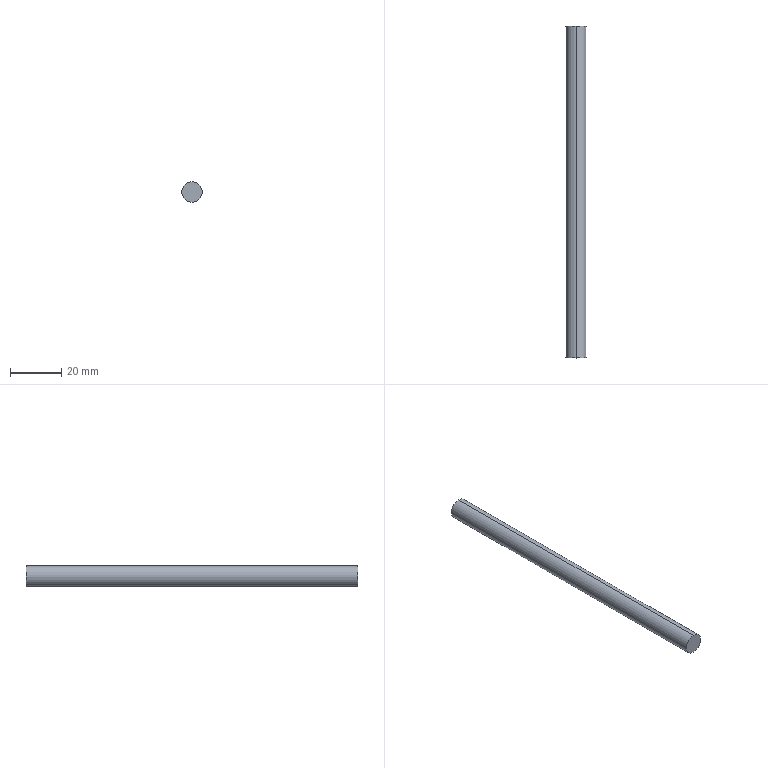Component | SolidWorks | LeadScrewM8x130-1 | 1 solid | 4 faces | box 8 x 130 x 8 mm | volume 6535 mm3 | cylinder 2 | plane 2 | commonest cylinder face diameters 8 x2
STEP:
#1=COLOUR_RGB('',0.7922,0.8196,0.9333);
#2=FILL_AREA_STYLE_COLOUR('',#1);
#3=FILL_AREA_STYLE('',(#2));
#4=SURFACE_STYLE_FILL_AREA(#3);
#5=SURFACE_SIDE_STYLE('',(#4));
#6=SURFACE_STYLE_USAGE(.BOTH.,#5);
#7=PRESENTATION_STYLE_ASSIGNMENT((#6));
#8=CARTESIAN_POINT('',(240.374,117.231,2.023));
#9=VERTEX_POINT('',#8);
#10=CARTESIAN_POINT('',(240.374,117.231,1.708));
#11=VERTEX_POINT('',#10);
#12=CARTESIAN_POINT('',(240.374,117.231,1.865));
#13=DIRECTION('',(0.,1.,-0.));
#14=DIRECTION('',(0.,0.,-1.));
#15=AXIS2_PLACEMENT_3D('',#12,#13,#14);
#16=CIRCLE('',#15,0.1575);
#17=EDGE_CURVE('',#9,#11,#16,.T.);
#18=ORIENTED_EDGE('',*,*,#17,.T.);
#19=CARTESIAN_POINT('',(240.374,122.35,1.708));
#20=VERTEX_POINT('',#19);
#21=CARTESIAN_POINT('',(240.374,118.413,1.708));
#22=DIRECTION('',(0.,1.,-0.));
#23=VECTOR('',#22,39.37);
#24=LINE('',#21,#23);
#25=EDGE_CURVE('',#11,#20,#24,.T.);
#26=ORIENTED_EDGE('',*,*,#25,.T.);
#27=CARTESIAN_POINT('',(240.374,122.35,2.023));
#28=VERTEX_POINT('',#27);
#29=CARTESIAN_POINT('',(240.374,122.35,1.865));
#30=DIRECTION('',(-0.,-1.,0.));
#31=DIRECTION('',(0.,0.,-1.));
#32=AXIS2_PLACEMENT_3D('',#29,#30,#31);
#33=CIRCLE('',#32,0.1575);
#34=EDGE_CURVE('',#20,#28,#33,.T.);
#35=ORIENTED_EDGE('',*,*,#34,.T.);
#36=CARTESIAN_POINT('',(240.374,118.413,2.023));
#37=DIRECTION('',(0.,1.,-0.));
#38=VECTOR('',#37,39.37);
#39=LINE('',#36,#38);
#40=EDGE_CURVE('',#9,#28,#39,.T.);
#41=ORIENTED_EDGE('',*,*,#40,.F.);
#42=EDGE_LOOP('',(#18,#26,#35,#41));
#43=FACE_OUTER_BOUND('',#42,.T.);
#44=CARTESIAN_POINT('',(240.374,118.413,1.865));
#45=DIRECTION('',(0.,1.,-0.));
#46=DIRECTION('',(0.,0.,1.));
#47=AXIS2_PLACEMENT_3D('',#44,#45,#46);
#48=CYLINDRICAL_SURFACE('',#47,0.1575);
#49=ADVANCED_FACE('',(#43),#48,.T.);
#50=CARTESIAN_POINT('',(240.374,122.35,1.865));
#51=DIRECTION('',(-0.,-1.,0.));
#52=DIRECTION('',(0.,0.,-1.));
#53=AXIS2_PLACEMENT_3D('',#50,#51,#52);
#54=CIRCLE('',#53,0.1575);
#55=EDGE_CURVE('',#28,#20,#54,.T.);
#56=ORIENTED_EDGE('',*,*,#55,.F.);
#57=ORIENTED_EDGE('',*,*,#34,.F.);
#58=EDGE_LOOP('',(#56,#57));
#59=FACE_OUTER_BOUND('',#58,.T.);
#60=CARTESIAN_POINT('',(240.374,122.35,1.865));
#61=DIRECTION('',(0.,1.,0.));
#62=DIRECTION('',(0.,0.,1.));
#63=AXIS2_PLACEMENT_3D('',#60,#61,#62);
#64=PLANE('',#63);
#65=ADVANCED_FACE('',(#59),#64,.T.);
#66=ORIENTED_EDGE('',*,*,#17,.F.);
#67=CARTESIAN_POINT('',(240.374,117.231,1.865));
#68=DIRECTION('',(0.,1.,-0.));
#69=DIRECTION('',(0.,0.,-1.));
#70=AXIS2_PLACEMENT_3D('',#67,#68,#69);
#71=CIRCLE('',#70,0.1575);
#72=EDGE_CURVE('',#11,#9,#71,.T.);
#73=ORIENTED_EDGE('',*,*,#72,.F.);
#74=EDGE_LOOP('',(#66,#73));
#75=FACE_OUTER_BOUND('',#74,.T.);
#76=CARTESIAN_POINT('',(240.374,117.231,1.865));
#77=DIRECTION('',(-0.,-1.,0.));
#78=DIRECTION('',(0.,0.,-1.));
#79=AXIS2_PLACEMENT_3D('',#76,#77,#78);
#80=PLANE('',#79);
#81=ADVANCED_FACE('',(#75),#80,.T.);
#82=ORIENTED_EDGE('',*,*,#25,.F.);
#83=ORIENTED_EDGE('',*,*,#72,.T.);
#84=ORIENTED_EDGE('',*,*,#40,.T.);
#85=ORIENTED_EDGE('',*,*,#55,.T.);
#86=EDGE_LOOP('',(#82,#83,#84,#85));
#87=FACE_OUTER_BOUND('',#86,.T.);
#88=CARTESIAN_POINT('',(240.374,118.413,1.865));
#89=DIRECTION('',(0.,1.,-0.));
#90=DIRECTION('',(0.,0.,1.));
#91=AXIS2_PLACEMENT_3D('',#88,#89,#90);
#92=CYLINDRICAL_SURFACE('',#91,0.1575);
#93=ADVANCED_FACE('',(#87),#92,.T.);
#94=CLOSED_SHELL('',(#49,#65,#81,#93));
#95=MANIFOLD_SOLID_BREP('',#94);
#96=STYLED_ITEM('',(#7),#95);
#97=PRESENTATION_LAYER_ASSIGNMENT('','',(#96));
#98=(LENGTH_UNIT()NAMED_UNIT(*)SI_UNIT($,.METRE.));
#99=LENGTH_MEASURE_WITH_UNIT(LENGTH_MEASURE(0.0254),#98);
#100=DIMENSIONAL_EXPONENTS(1.,0.,0.,0.,0.,0.,0.);
#101=(CONVERSION_BASED_UNIT('',#99)LENGTH_UNIT()NAMED_UNIT(#100));
#102=UNCERTAINTY_MEASURE_WITH_UNIT(LENGTH_MEASURE(0.00001),#101,'','');
#103=(NAMED_UNIT(*)PLANE_ANGLE_UNIT()SI_UNIT($,.RADIAN.));
#104=(NAMED_UNIT(*)SI_UNIT($,.STERADIAN.)SOLID_ANGLE_UNIT());
#105=(GEOMETRIC_REPRESENTATION_CONTEXT(3)GLOBAL_UNCERTAINTY_ASSIGNED_CONTEXT((#102))GLOBAL_UNIT_ASSIGNED_CONTEXT((#101,#103,#104))REPRESENTATION_CONTEXT('',''));
#106=MECHANICAL_DESIGN_GEOMETRIC_PRESENTATION_REPRESENTATION('',(#96),#105);
#107=CARTESIAN_POINT('',(0.,0.,0.));
#108=DIRECTION('',(0.,0.,1.));
#109=DIRECTION('',(1.,0.,0.));
#110=AXIS2_PLACEMENT_3D('',#107,#108,#109);
#111=(LENGTH_UNIT()NAMED_UNIT(*)SI_UNIT($,.METRE.));
#112=LENGTH_MEASURE_WITH_UNIT(LENGTH_MEASURE(0.0254),#111);
#113=DIMENSIONAL_EXPONENTS(1.,0.,0.,0.,0.,0.,0.);
#114=(CONVERSION_BASED_UNIT('',#112)LENGTH_UNIT()NAMED_UNIT(#113));
#115=UNCERTAINTY_MEASURE_WITH_UNIT(LENGTH_MEASURE(0.00001),#114,'','');
#116=(NAMED_UNIT(*)PLANE_ANGLE_UNIT()SI_UNIT($,.RADIAN.));
#117=(NAMED_UNIT(*)SI_UNIT($,.STERADIAN.)SOLID_ANGLE_UNIT());
#118=(GEOMETRIC_REPRESENTATION_CONTEXT(3)GLOBAL_UNCERTAINTY_ASSIGNED_CONTEXT((#115))GLOBAL_UNIT_ASSIGNED_CONTEXT((#114,#116,#117))REPRESENTATION_CONTEXT('',''));
#119=ADVANCED_BREP_SHAPE_REPRESENTATION('',(#95,#110),#118);